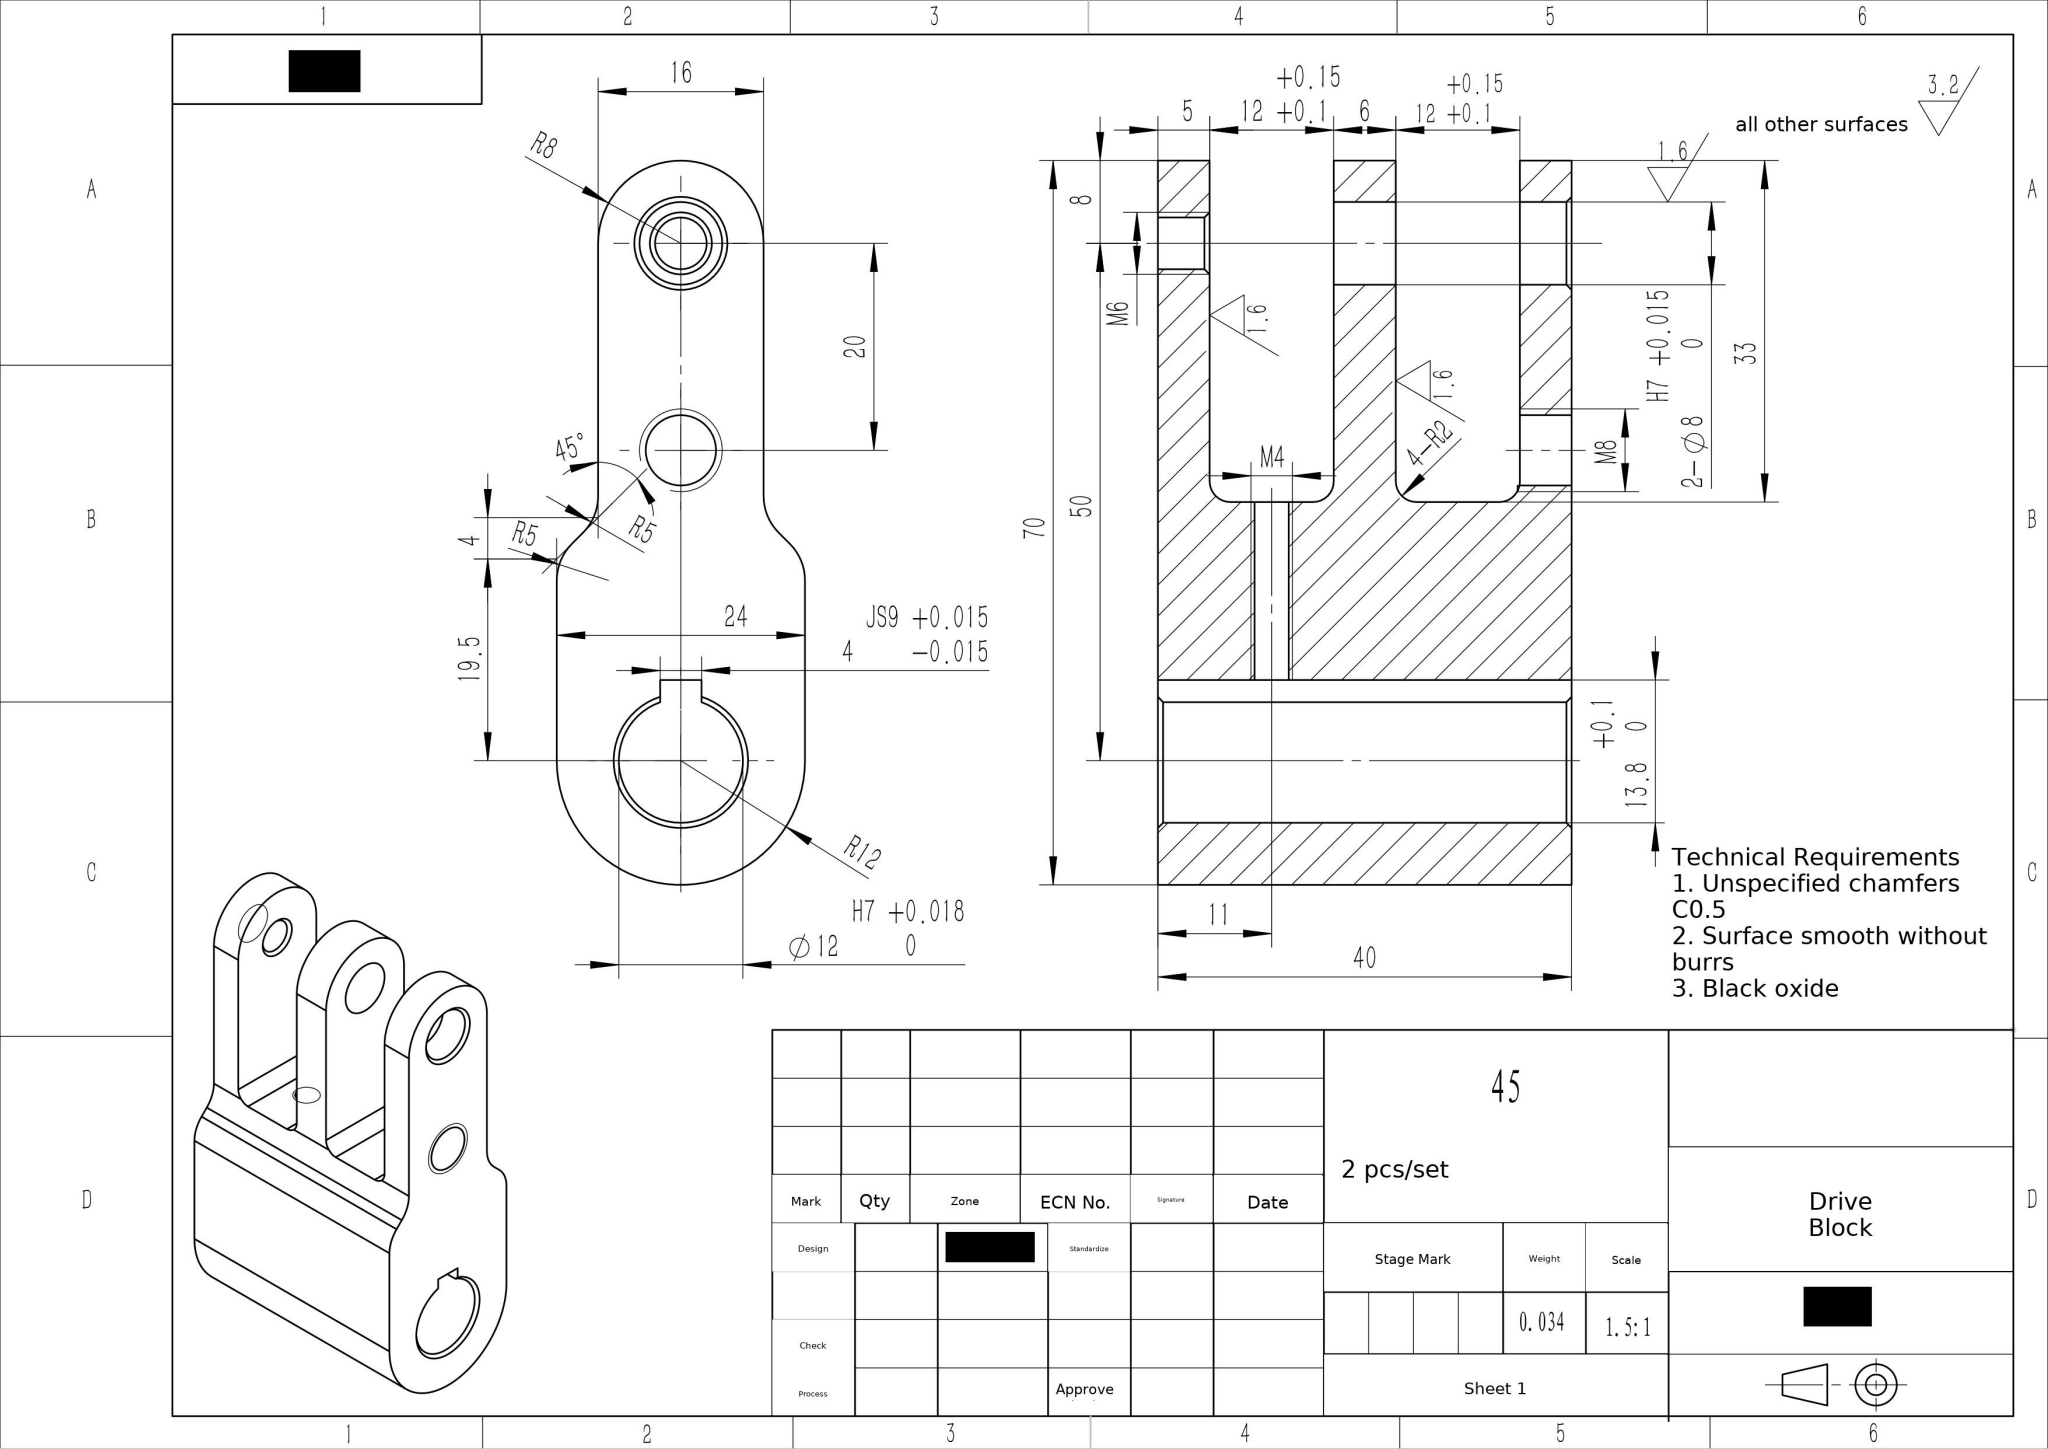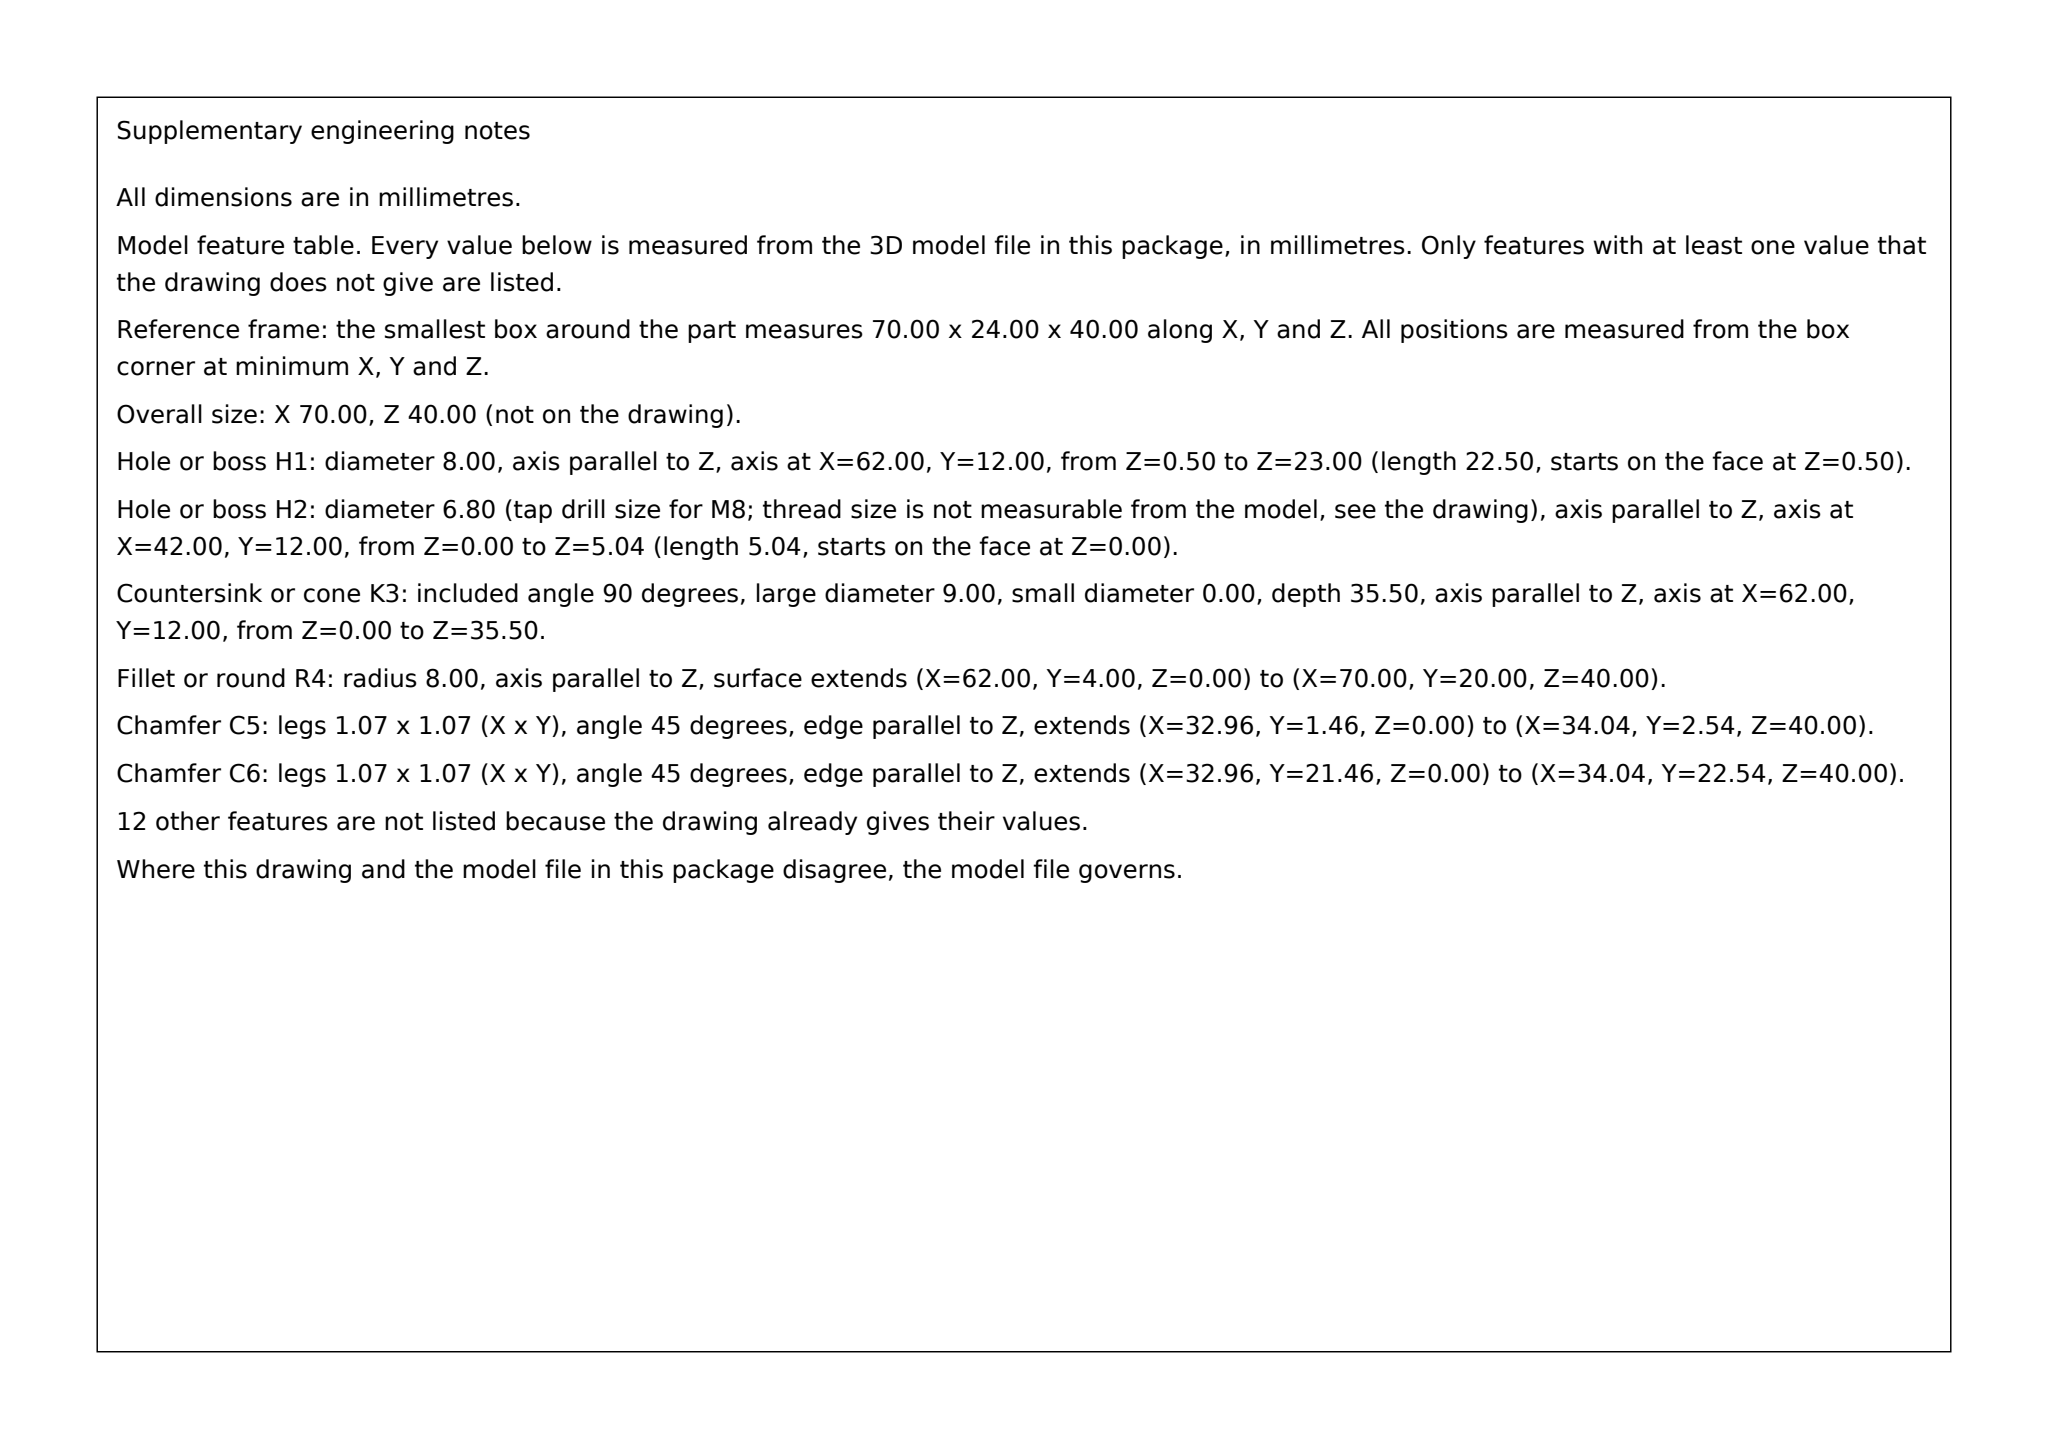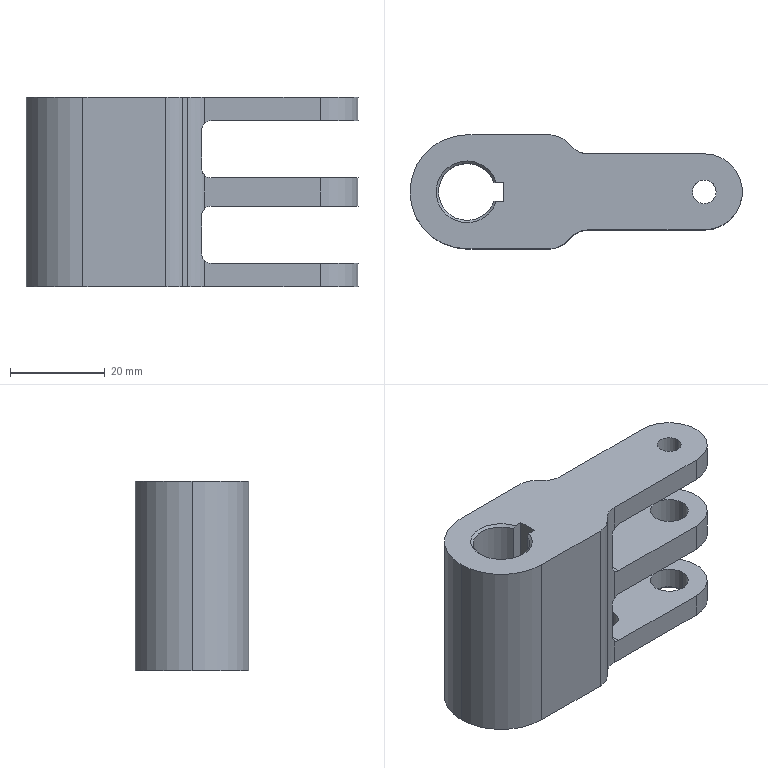Part | SolidWorks | mm | material 45 | 1 solid | 53 faces | box 70 x 24 x 40 mm | volume 34167 mm3 | cylinder 25 | plane 21 | cone 7 | commonest cylinder face diameters 8 x4 10 x4 4 x4 16 x3 6.8 x2 5 x2 3.3 x2 12 x2